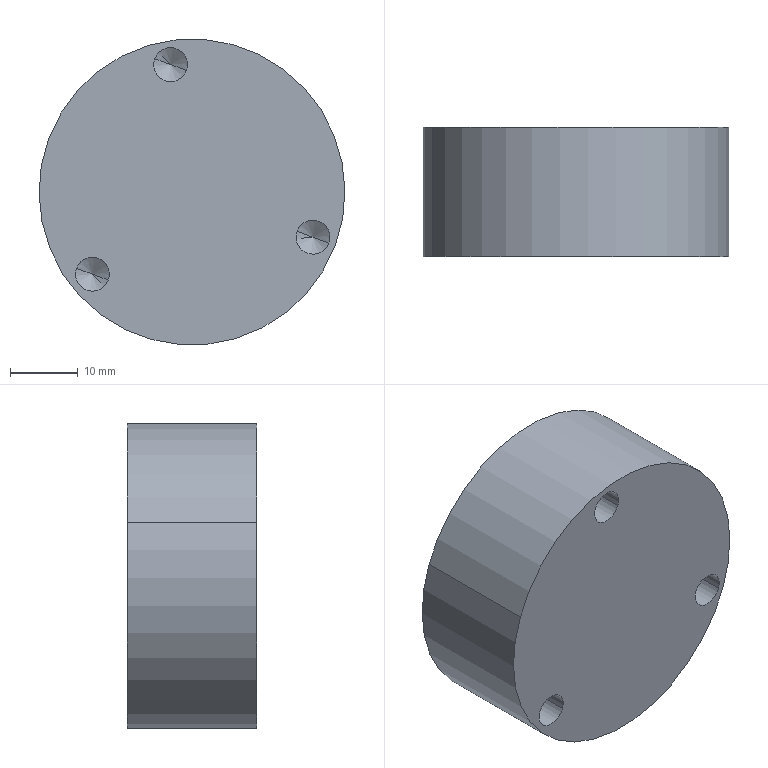Component | SolidWorks | BearingBlock-1 | 1 solid | 20 faces | box 45 x 19 x 45 mm | volume 18714 mm3 | cylinder 10 | cone 6 | spline 2 | plane 2 | commonest cylinder face diameters 5 x6 36.33 x2 45 x2
STEP:
#1=COLOUR_RGB('',0.7922,0.8196,0.9333);
#2=FILL_AREA_STYLE_COLOUR('',#1);
#3=FILL_AREA_STYLE('',(#2));
#4=SURFACE_STYLE_FILL_AREA(#3);
#5=SURFACE_SIDE_STYLE('',(#4));
#6=SURFACE_STYLE_USAGE(.BOTH.,#5);
#7=PRESENTATION_STYLE_ASSIGNMENT((#6));
#8=CARTESIAN_POINT('',(3.722,1.024,19.608));
#9=VERTEX_POINT('',#8);
#10=CARTESIAN_POINT('',(5.061,1.024,19.107));
#11=VERTEX_POINT('',#10);
#12=CARTESIAN_POINT('',(4.392,1.024,19.357));
#13=DIRECTION('',(-0.,1.,0.));
#14=DIRECTION('',(-0.9367,-0.,0.3501));
#15=AXIS2_PLACEMENT_3D('',#12,#13,#14);
#16=CIRCLE('',#15,0.7152);
#17=EDGE_CURVE('',#9,#11,#16,.T.);
#18=ORIENTED_EDGE('',*,*,#17,.T.);
#19=CARTESIAN_POINT('',(4.392,0.5906,19.357));
#20=VERTEX_POINT('',#19);
#21=CARTESIAN_POINT('',(5.061,1.024,19.107));
#22=CARTESIAN_POINT('',(4.727,0.5905,19.232));
#23=CARTESIAN_POINT('',(4.392,0.5906,19.357));
#24=B_SPLINE_CURVE_WITH_KNOTS('',2,(#21,#22,#23),.UNSPECIFIED.,.F.,.F.,(3,3),(0.06428,0.5001),.UNSPECIFIED.);
#25=EDGE_CURVE('',#11,#20,#24,.T.);
#26=ORIENTED_EDGE('',*,*,#25,.T.);
#27=CARTESIAN_POINT('',(3.722,1.024,19.608));
#28=CARTESIAN_POINT('',(4.057,0.5905,19.482));
#29=CARTESIAN_POINT('',(4.392,0.5906,19.357));
#30=B_SPLINE_CURVE_WITH_KNOTS('',2,(#27,#28,#29),.UNSPECIFIED.,.F.,.F.,(3,3),(0.06428,0.5001),.UNSPECIFIED.);
#31=EDGE_CURVE('',#9,#20,#30,.T.);
#32=ORIENTED_EDGE('',*,*,#31,.F.);
#33=EDGE_LOOP('',(#18,#26,#32));
#34=FACE_OUTER_BOUND('',#33,.T.);
#35=CARTESIAN_POINT('',(3.722,1.024,19.608));
#36=CARTESIAN_POINT('',(4.222,1.024,20.947));
#37=CARTESIAN_POINT('',(5.562,1.024,20.447));
#38=CARTESIAN_POINT('',(5.061,1.024,19.107));
#39=CARTESIAN_POINT('',(4.057,0.5905,19.482));
#40=CARTESIAN_POINT('',(4.307,0.5905,20.152));
#41=CARTESIAN_POINT('',(4.977,0.5905,19.902));
#42=CARTESIAN_POINT('',(4.727,0.5905,19.232));
#43=CARTESIAN_POINT('',(4.392,0.5906,19.357));
#44=CARTESIAN_POINT('',(4.392,0.5906,19.357));
#45=CARTESIAN_POINT('',(4.392,0.5906,19.357));
#46=CARTESIAN_POINT('',(4.392,0.5906,19.357));
#47=(BOUNDED_SURFACE()B_SPLINE_SURFACE(2,3,((#35,#36,#37,#38),(#39,#40,#41,#42),(#43,#44,#45,#46)),.UNSPECIFIED.,.F.,.F.,.F.)B_SPLINE_SURFACE_WITH_KNOTS((3,3),(4,4),(0.06428,0.5001),(0.,1.),.UNSPECIFIED.)GEOMETRIC_REPRESENTATION_ITEM()RATIONAL_B_SPLINE_SURFACE(((1.,0.3333,0.3333,1.),(1.,0.3333,0.3333,1.),(1.,0.3333,0.3333,1.)))REPRESENTATION_ITEM('')SURFACE());
#48=ADVANCED_FACE('',(#34),#47,.F.);
#49=CARTESIAN_POINT('',(4.176,0.8661,20.129));
#50=VERTEX_POINT('',#49);
#51=CARTESIAN_POINT('',(4.36,0.8661,20.06));
#52=VERTEX_POINT('',#51);
#53=CARTESIAN_POINT('',(4.268,0.8661,20.095));
#54=DIRECTION('',(0.,-1.,-0.));
#55=DIRECTION('',(0.9367,0.,-0.3501));
#56=AXIS2_PLACEMENT_3D('',#53,#54,#55);
#57=CIRCLE('',#56,0.09843);
#58=EDGE_CURVE('',#50,#52,#57,.T.);
#59=ORIENTED_EDGE('',*,*,#58,.F.);
#60=CARTESIAN_POINT('',(4.176,0.4724,20.129));
#61=VERTEX_POINT('',#60);
#62=CARTESIAN_POINT('',(4.176,0.4724,20.129));
#63=DIRECTION('',(0.,-1.,-0.));
#64=VECTOR('',#63,39.37);
#65=LINE('',#62,#64);
#66=EDGE_CURVE('',#50,#61,#65,.T.);
#67=ORIENTED_EDGE('',*,*,#66,.T.);
#68=CARTESIAN_POINT('',(4.36,0.4724,20.06));
#69=VERTEX_POINT('',#68);
#70=CARTESIAN_POINT('',(4.268,0.4724,20.095));
#71=DIRECTION('',(0.,-1.,-0.));
#72=DIRECTION('',(0.9367,0.,-0.3501));
#73=AXIS2_PLACEMENT_3D('',#70,#71,#72);
#74=CIRCLE('',#73,0.09843);
#75=EDGE_CURVE('',#61,#69,#74,.T.);
#76=ORIENTED_EDGE('',*,*,#75,.T.);
#77=CARTESIAN_POINT('',(4.36,0.4724,20.06));
#78=DIRECTION('',(0.,-1.,-0.));
#79=VECTOR('',#78,39.37);
#80=LINE('',#77,#79);
#81=EDGE_CURVE('',#52,#69,#80,.T.);
#82=ORIENTED_EDGE('',*,*,#81,.F.);
#83=EDGE_LOOP('',(#59,#67,#76,#82));
#84=FACE_OUTER_BOUND('',#83,.T.);
#85=CARTESIAN_POINT('',(4.268,0.4724,20.095));
#86=DIRECTION('',(0.,-1.,-0.));
#87=DIRECTION('',(0.9367,0.,-0.3501));
#88=AXIS2_PLACEMENT_3D('',#85,#86,#87);
#89=CYLINDRICAL_SURFACE('',#88,0.09843);
#90=ADVANCED_FACE('',(#84),#89,.F.);
#91=CARTESIAN_POINT('',(4.268,0.9253,20.095));
#92=VERTEX_POINT('',#91);
#93=CARTESIAN_POINT('',(4.36,0.8661,20.06));
#94=DIRECTION('',(0.8029,-0.515,-0.3001));
#95=VECTOR('',#94,39.37);
#96=LINE('',#93,#95);
#97=EDGE_CURVE('',#92,#52,#96,.T.);
#98=ORIENTED_EDGE('',*,*,#97,.F.);
#99=CARTESIAN_POINT('',(4.176,0.8661,20.129));
#100=DIRECTION('',(-0.8029,-0.515,0.3001));
#101=VECTOR('',#100,39.37);
#102=LINE('',#99,#101);
#103=EDGE_CURVE('',#92,#50,#102,.T.);
#104=ORIENTED_EDGE('',*,*,#103,.T.);
#105=ORIENTED_EDGE('',*,*,#58,.T.);
#106=EDGE_LOOP('',(#98,#104,#105));
#107=FACE_OUTER_BOUND('',#106,.T.);
#108=CARTESIAN_POINT('',(4.268,0.8661,20.095));
#109=DIRECTION('',(0.,-1.,-0.));
#110=DIRECTION('',(0.9367,0.,-0.3501));
#111=AXIS2_PLACEMENT_3D('',#108,#109,#110);
#112=CONICAL_SURFACE('',#111,0.09843,1.03);
#113=ADVANCED_FACE('',(#107),#112,.F.);
#114=CARTESIAN_POINT('',(5.,0.8661,19.13));
#115=VERTEX_POINT('',#114);
#116=CARTESIAN_POINT('',(5.184,0.8661,19.061));
#117=VERTEX_POINT('',#116);
#118=CARTESIAN_POINT('',(5.092,0.8661,19.095));
#119=DIRECTION('',(0.,-1.,-0.));
#120=DIRECTION('',(0.9367,0.,-0.3501));
#121=AXIS2_PLACEMENT_3D('',#118,#119,#120);
#122=CIRCLE('',#121,0.09843);
#123=EDGE_CURVE('',#115,#117,#122,.T.);
#124=ORIENTED_EDGE('',*,*,#123,.F.);
#125=CARTESIAN_POINT('',(5.,0.4724,19.13));
#126=VERTEX_POINT('',#125);
#127=CARTESIAN_POINT('',(5.,0.4724,19.13));
#128=DIRECTION('',(0.,-1.,-0.));
#129=VECTOR('',#128,39.37);
#130=LINE('',#127,#129);
#131=EDGE_CURVE('',#115,#126,#130,.T.);
#132=ORIENTED_EDGE('',*,*,#131,.T.);
#133=CARTESIAN_POINT('',(5.184,0.4724,19.061));
#134=VERTEX_POINT('',#133);
#135=CARTESIAN_POINT('',(5.092,0.4724,19.095));
#136=DIRECTION('',(0.,-1.,-0.));
#137=DIRECTION('',(0.9367,0.,-0.3501));
#138=AXIS2_PLACEMENT_3D('',#135,#136,#137);
#139=CIRCLE('',#138,0.09843);
#140=EDGE_CURVE('',#126,#134,#139,.T.);
#141=ORIENTED_EDGE('',*,*,#140,.T.);
#142=CARTESIAN_POINT('',(5.184,0.4724,19.061));
#143=DIRECTION('',(0.,-1.,-0.));
#144=VECTOR('',#143,39.37);
#145=LINE('',#142,#144);
#146=EDGE_CURVE('',#117,#134,#145,.T.);
#147=ORIENTED_EDGE('',*,*,#146,.F.);
#148=EDGE_LOOP('',(#124,#132,#141,#147));
#149=FACE_OUTER_BOUND('',#148,.T.);
#150=CARTESIAN_POINT('',(5.092,0.4724,19.095));
#151=DIRECTION('',(0.,-1.,-0.));
#152=DIRECTION('',(0.9367,0.,-0.3501));
#153=AXIS2_PLACEMENT_3D('',#150,#151,#152);
#154=CYLINDRICAL_SURFACE('',#153,0.09843);
#155=ADVANCED_FACE('',(#149),#154,.F.);
#156=CARTESIAN_POINT('',(5.092,0.9253,19.095));
#157=VERTEX_POINT('',#156);
#158=CARTESIAN_POINT('',(5.184,0.8661,19.061));
#159=DIRECTION('',(0.8029,-0.515,-0.3001));
#160=VECTOR('',#159,39.37);
#161=LINE('',#158,#160);
#162=EDGE_CURVE('',#157,#117,#161,.T.);
#163=ORIENTED_EDGE('',*,*,#162,.F.);
#164=CARTESIAN_POINT('',(5.,0.8661,19.13));
#165=DIRECTION('',(-0.8029,-0.515,0.3001));
#166=VECTOR('',#165,39.37);
#167=LINE('',#164,#166);
#168=EDGE_CURVE('',#157,#115,#167,.T.);
#169=ORIENTED_EDGE('',*,*,#168,.T.);
#170=ORIENTED_EDGE('',*,*,#123,.T.);
#171=EDGE_LOOP('',(#163,#169,#170));
#172=FACE_OUTER_BOUND('',#171,.T.);
#173=CARTESIAN_POINT('',(5.092,0.8661,19.095));
#174=DIRECTION('',(0.,-1.,-0.));
#175=DIRECTION('',(0.9367,0.,-0.3501));
#176=AXIS2_PLACEMENT_3D('',#173,#174,#175);
#177=CONICAL_SURFACE('',#176,0.09843,1.03);
#178=ADVANCED_FACE('',(#172),#177,.F.);
#179=CARTESIAN_POINT('',(3.722,0.8661,18.916));
#180=VERTEX_POINT('',#179);
#181=CARTESIAN_POINT('',(3.907,0.8661,18.847));
#182=VERTEX_POINT('',#181);
#183=CARTESIAN_POINT('',(3.814,0.8661,18.881));
#184=DIRECTION('',(0.,-1.,-0.));
#185=DIRECTION('',(0.9367,0.,-0.3501));
#186=AXIS2_PLACEMENT_3D('',#183,#184,#185);
#187=CIRCLE('',#186,0.09843);
#188=EDGE_CURVE('',#180,#182,#187,.T.);
#189=ORIENTED_EDGE('',*,*,#188,.F.);
#190=CARTESIAN_POINT('',(3.722,0.4724,18.916));
#191=VERTEX_POINT('',#190);
#192=CARTESIAN_POINT('',(3.722,0.4724,18.916));
#193=DIRECTION('',(0.,-1.,-0.));
#194=VECTOR('',#193,39.37);
#195=LINE('',#192,#194);
#196=EDGE_CURVE('',#180,#191,#195,.T.);
#197=ORIENTED_EDGE('',*,*,#196,.T.);
#198=CARTESIAN_POINT('',(3.907,0.4724,18.847));
#199=VERTEX_POINT('',#198);
#200=CARTESIAN_POINT('',(3.814,0.4724,18.881));
#201=DIRECTION('',(0.,-1.,-0.));
#202=DIRECTION('',(0.9367,0.,-0.3501));
#203=AXIS2_PLACEMENT_3D('',#200,#201,#202);
#204=CIRCLE('',#203,0.09843);
#205=EDGE_CURVE('',#191,#199,#204,.T.);
#206=ORIENTED_EDGE('',*,*,#205,.T.);
#207=CARTESIAN_POINT('',(3.907,0.4724,18.847));
#208=DIRECTION('',(0.,-1.,-0.));
#209=VECTOR('',#208,39.37);
#210=LINE('',#207,#209);
#211=EDGE_CURVE('',#182,#199,#210,.T.);
#212=ORIENTED_EDGE('',*,*,#211,.F.);
#213=EDGE_LOOP('',(#189,#197,#206,#212));
#214=FACE_OUTER_BOUND('',#213,.T.);
#215=CARTESIAN_POINT('',(3.814,0.4724,18.881));
#216=DIRECTION('',(0.,-1.,-0.));
#217=DIRECTION('',(0.9367,0.,-0.3501));
#218=AXIS2_PLACEMENT_3D('',#215,#216,#217);
#219=CYLINDRICAL_SURFACE('',#218,0.09843);
#220=ADVANCED_FACE('',(#214),#219,.F.);
#221=CARTESIAN_POINT('',(3.814,0.9253,18.881));
#222=VERTEX_POINT('',#221);
#223=CARTESIAN_POINT('',(3.907,0.8661,18.847));
#224=DIRECTION('',(0.8029,-0.515,-0.3001));
#225=VECTOR('',#224,39.37);
#226=LINE('',#223,#225);
#227=EDGE_CURVE('',#222,#182,#226,.T.);
#228=ORIENTED_EDGE('',*,*,#227,.F.);
#229=CARTESIAN_POINT('',(3.722,0.8661,18.916));
#230=DIRECTION('',(-0.8029,-0.515,0.3001));
#231=VECTOR('',#230,39.37);
#232=LINE('',#229,#231);
#233=EDGE_CURVE('',#222,#180,#232,.T.);
#234=ORIENTED_EDGE('',*,*,#233,.T.);
#235=ORIENTED_EDGE('',*,*,#188,.T.);
#236=EDGE_LOOP('',(#228,#234,#235));
#237=FACE_OUTER_BOUND('',#236,.T.);
#238=CARTESIAN_POINT('',(3.814,0.8661,18.881));
#239=DIRECTION('',(0.,-1.,-0.));
#240=DIRECTION('',(0.9367,0.,-0.3501));
#241=AXIS2_PLACEMENT_3D('',#238,#239,#240);
#242=CONICAL_SURFACE('',#241,0.09843,1.03);
#243=ADVANCED_FACE('',(#237),#242,.F.);
#244=CARTESIAN_POINT('',(4.392,1.024,19.357));
#245=DIRECTION('',(-0.,1.,0.));
#246=DIRECTION('',(-0.9367,-0.,0.3501));
#247=AXIS2_PLACEMENT_3D('',#244,#245,#246);
#248=CIRCLE('',#247,0.7152);
#249=EDGE_CURVE('',#11,#9,#248,.T.);
#250=ORIENTED_EDGE('',*,*,#249,.F.);
#251=CARTESIAN_POINT('',(5.061,1.22,19.107));
#252=VERTEX_POINT('',#251);
#253=CARTESIAN_POINT('',(5.061,1.024,19.107));
#254=DIRECTION('',(-0.,1.,0.));
#255=VECTOR('',#254,39.37);
#256=LINE('',#253,#255);
#257=EDGE_CURVE('',#11,#252,#256,.T.);
#258=ORIENTED_EDGE('',*,*,#257,.T.);
#259=CARTESIAN_POINT('',(3.722,1.22,19.608));
#260=VERTEX_POINT('',#259);
#261=CARTESIAN_POINT('',(4.392,1.22,19.357));
#262=DIRECTION('',(-0.,1.,0.));
#263=DIRECTION('',(-0.9367,-0.,0.3501));
#264=AXIS2_PLACEMENT_3D('',#261,#262,#263);
#265=CIRCLE('',#264,0.7152);
#266=EDGE_CURVE('',#252,#260,#265,.T.);
#267=ORIENTED_EDGE('',*,*,#266,.T.);
#268=CARTESIAN_POINT('',(3.722,1.024,19.608));
#269=DIRECTION('',(-0.,1.,0.));
#270=VECTOR('',#269,39.37);
#271=LINE('',#268,#270);
#272=EDGE_CURVE('',#9,#260,#271,.T.);
#273=ORIENTED_EDGE('',*,*,#272,.F.);
#274=EDGE_LOOP('',(#250,#258,#267,#273));
#275=FACE_OUTER_BOUND('',#274,.T.);
#276=CARTESIAN_POINT('',(4.392,1.024,19.357));
#277=DIRECTION('',(-0.,1.,0.));
#278=DIRECTION('',(-0.9367,-0.,0.3501));
#279=AXIS2_PLACEMENT_3D('',#276,#277,#278);
#280=CYLINDRICAL_SURFACE('',#279,0.7152);
#281=ADVANCED_FACE('',(#275),#280,.F.);
#282=CARTESIAN_POINT('',(5.221,1.22,19.047));
#283=VERTEX_POINT('',#282);
#284=CARTESIAN_POINT('',(3.562,1.22,19.667));
#285=VERTEX_POINT('',#284);
#286=CARTESIAN_POINT('',(4.392,1.22,19.357));
#287=DIRECTION('',(0.,-1.,-0.));
#288=DIRECTION('',(0.9367,0.,-0.3501));
#289=AXIS2_PLACEMENT_3D('',#286,#287,#288);
#290=CIRCLE('',#289,0.8858);
#291=EDGE_CURVE('',#283,#285,#290,.T.);
#292=ORIENTED_EDGE('',*,*,#291,.T.);
#293=CARTESIAN_POINT('',(3.562,0.4724,19.667));
#294=VERTEX_POINT('',#293);
#295=CARTESIAN_POINT('',(3.562,1.22,19.667));
#296=DIRECTION('',(0.,-1.,-0.));
#297=VECTOR('',#296,39.37);
#298=LINE('',#295,#297);
#299=EDGE_CURVE('',#285,#294,#298,.T.);
#300=ORIENTED_EDGE('',*,*,#299,.T.);
#301=CARTESIAN_POINT('',(5.221,0.4724,19.047));
#302=VERTEX_POINT('',#301);
#303=CARTESIAN_POINT('',(4.392,0.4724,19.357));
#304=DIRECTION('',(0.,-1.,-0.));
#305=DIRECTION('',(0.9367,0.,-0.3501));
#306=AXIS2_PLACEMENT_3D('',#303,#304,#305);
#307=CIRCLE('',#306,0.8858);
#308=EDGE_CURVE('',#302,#294,#307,.T.);
#309=ORIENTED_EDGE('',*,*,#308,.F.);
#310=CARTESIAN_POINT('',(5.221,1.22,19.047));
#311=DIRECTION('',(0.,-1.,-0.));
#312=VECTOR('',#311,39.37);
#313=LINE('',#310,#312);
#314=EDGE_CURVE('',#283,#302,#313,.T.);
#315=ORIENTED_EDGE('',*,*,#314,.F.);
#316=EDGE_LOOP('',(#292,#300,#309,#315));
#317=FACE_OUTER_BOUND('',#316,.T.);
#318=CARTESIAN_POINT('',(4.392,1.22,19.357));
#319=DIRECTION('',(0.,-1.,-0.));
#320=DIRECTION('',(0.9367,0.,-0.3501));
#321=AXIS2_PLACEMENT_3D('',#318,#319,#320);
#322=CYLINDRICAL_SURFACE('',#321,0.8858);
#323=ADVANCED_FACE('',(#317),#322,.T.);
#324=ORIENTED_EDGE('',*,*,#299,.F.);
#325=CARTESIAN_POINT('',(4.392,1.22,19.357));
#326=DIRECTION('',(0.,-1.,-0.));
#327=DIRECTION('',(0.9367,0.,-0.3501));
#328=AXIS2_PLACEMENT_3D('',#325,#326,#327);
#329=CIRCLE('',#328,0.8858);
#330=EDGE_CURVE('',#285,#283,#329,.T.);
#331=ORIENTED_EDGE('',*,*,#330,.T.);
#332=ORIENTED_EDGE('',*,*,#314,.T.);
#333=CARTESIAN_POINT('',(4.392,0.4724,19.357));
#334=DIRECTION('',(0.,-1.,-0.));
#335=DIRECTION('',(0.9367,0.,-0.3501));
#336=AXIS2_PLACEMENT_3D('',#333,#334,#335);
#337=CIRCLE('',#336,0.8858);
#338=EDGE_CURVE('',#294,#302,#337,.T.);
#339=ORIENTED_EDGE('',*,*,#338,.F.);
#340=EDGE_LOOP('',(#324,#331,#332,#339));
#341=FACE_OUTER_BOUND('',#340,.T.);
#342=CARTESIAN_POINT('',(4.392,1.22,19.357));
#343=DIRECTION('',(0.,-1.,-0.));
#344=DIRECTION('',(0.9367,0.,-0.3501));
#345=AXIS2_PLACEMENT_3D('',#342,#343,#344);
#346=CYLINDRICAL_SURFACE('',#345,0.8858);
#347=ADVANCED_FACE('',(#341),#346,.T.);
#348=CARTESIAN_POINT('',(4.392,1.22,19.357));
#349=DIRECTION('',(-0.,1.,0.));
#350=DIRECTION('',(-0.9367,-0.,0.3501));
#351=AXIS2_PLACEMENT_3D('',#348,#349,#350);
#352=CIRCLE('',#351,0.7152);
#353=EDGE_CURVE('',#260,#252,#352,.T.);
#354=ORIENTED_EDGE('',*,*,#353,.F.);
#355=ORIENTED_EDGE('',*,*,#266,.F.);
#356=EDGE_LOOP('',(#354,#355));
#357=FACE_BOUND('',#356,.T.);
#358=ORIENTED_EDGE('',*,*,#291,.F.);
#359=ORIENTED_EDGE('',*,*,#330,.F.);
#360=EDGE_LOOP('',(#358,#359));
#361=FACE_OUTER_BOUND('',#360,.T.);
#362=CARTESIAN_POINT('',(4.392,1.22,19.357));
#363=DIRECTION('',(0.,-1.,-0.));
#364=DIRECTION('',(0.9367,0.,-0.3501));
#365=AXIS2_PLACEMENT_3D('',#362,#363,#364);
#366=PLANE('',#365);
#367=ADVANCED_FACE('',(#357,#361),#366,.F.);
#368=CARTESIAN_POINT('',(4.268,0.4724,20.095));
#369=DIRECTION('',(0.,-1.,-0.));
#370=DIRECTION('',(0.9367,0.,-0.3501));
#371=AXIS2_PLACEMENT_3D('',#368,#369,#370);
#372=CIRCLE('',#371,0.09843);
#373=EDGE_CURVE('',#69,#61,#372,.T.);
#374=ORIENTED_EDGE('',*,*,#373,.F.);
#375=ORIENTED_EDGE('',*,*,#75,.F.);
#376=EDGE_LOOP('',(#374,#375));
#377=FACE_BOUND('',#376,.T.);
#378=CARTESIAN_POINT('',(5.092,0.4724,19.095));
#379=DIRECTION('',(0.,-1.,-0.));
#380=DIRECTION('',(0.9367,0.,-0.3501));
#381=AXIS2_PLACEMENT_3D('',#378,#379,#380);
#382=CIRCLE('',#381,0.09843);
#383=EDGE_CURVE('',#134,#126,#382,.T.);
#384=ORIENTED_EDGE('',*,*,#383,.F.);
#385=ORIENTED_EDGE('',*,*,#140,.F.);
#386=EDGE_LOOP('',(#384,#385));
#387=FACE_BOUND('',#386,.T.);
#388=CARTESIAN_POINT('',(3.814,0.4724,18.881));
#389=DIRECTION('',(0.,-1.,-0.));
#390=DIRECTION('',(0.9367,0.,-0.3501));
#391=AXIS2_PLACEMENT_3D('',#388,#389,#390);
#392=CIRCLE('',#391,0.09843);
#393=EDGE_CURVE('',#199,#191,#392,.T.);
#394=ORIENTED_EDGE('',*,*,#393,.F.);
#395=ORIENTED_EDGE('',*,*,#205,.F.);
#396=EDGE_LOOP('',(#394,#395));
#397=FACE_BOUND('',#396,.T.);
#398=ORIENTED_EDGE('',*,*,#308,.T.);
#399=ORIENTED_EDGE('',*,*,#338,.T.);
#400=EDGE_LOOP('',(#398,#399));
#401=FACE_OUTER_BOUND('',#400,.T.);
#402=CARTESIAN_POINT('',(4.392,0.4724,19.357));
#403=DIRECTION('',(0.,-1.,-0.));
#404=DIRECTION('',(0.9367,0.,-0.3501));
#405=AXIS2_PLACEMENT_3D('',#402,#403,#404);
#406=PLANE('',#405);
#407=ADVANCED_FACE('',(#377,#387,#397,#401),#406,.T.);
#408=ORIENTED_EDGE('',*,*,#257,.F.);
#409=ORIENTED_EDGE('',*,*,#17,.F.);
#410=ORIENTED_EDGE('',*,*,#272,.T.);
#411=ORIENTED_EDGE('',*,*,#353,.T.);
#412=EDGE_LOOP('',(#408,#409,#410,#411));
#413=FACE_OUTER_BOUND('',#412,.T.);
#414=CARTESIAN_POINT('',(4.392,1.024,19.357));
#415=DIRECTION('',(-0.,1.,0.));
#416=DIRECTION('',(-0.9367,-0.,0.3501));
#417=AXIS2_PLACEMENT_3D('',#414,#415,#416);
#418=CYLINDRICAL_SURFACE('',#417,0.7152);
#419=ADVANCED_FACE('',(#413),#418,.F.);
#420=ORIENTED_EDGE('',*,*,#25,.F.);
#421=ORIENTED_EDGE('',*,*,#249,.T.);
#422=ORIENTED_EDGE('',*,*,#31,.T.);
#423=EDGE_LOOP('',(#420,#421,#422));
#424=FACE_OUTER_BOUND('',#423,.T.);
#425=CARTESIAN_POINT('',(5.061,1.024,19.107));
#426=CARTESIAN_POINT('',(4.561,1.024,17.767));
#427=CARTESIAN_POINT('',(3.221,1.024,18.268));
#428=CARTESIAN_POINT('',(3.722,1.024,19.608));
#429=CARTESIAN_POINT('',(4.727,0.5905,19.232));
#430=CARTESIAN_POINT('',(4.476,0.5905,18.562));
#431=CARTESIAN_POINT('',(3.806,0.5905,18.812));
#432=CARTESIAN_POINT('',(4.057,0.5905,19.482));
#433=CARTESIAN_POINT('',(4.392,0.5906,19.357));
#434=CARTESIAN_POINT('',(4.392,0.5906,19.357));
#435=CARTESIAN_POINT('',(4.392,0.5906,19.357));
#436=CARTESIAN_POINT('',(4.392,0.5906,19.357));
#437=(BOUNDED_SURFACE()B_SPLINE_SURFACE(2,3,((#425,#426,#427,#428),(#429,#430,#431,#432),(#433,#434,#435,#436)),.UNSPECIFIED.,.F.,.F.,.F.)B_SPLINE_SURFACE_WITH_KNOTS((3,3),(4,4),(0.06428,0.5001),(0.,1.),.UNSPECIFIED.)GEOMETRIC_REPRESENTATION_ITEM()RATIONAL_B_SPLINE_SURFACE(((1.,0.3333,0.3333,1.),(1.,0.3333,0.3333,1.),(1.,0.3333,0.3333,1.)))REPRESENTATION_ITEM('')SURFACE());
#438=ADVANCED_FACE('',(#424),#437,.F.);
#439=ORIENTED_EDGE('',*,*,#233,.F.);
#440=ORIENTED_EDGE('',*,*,#227,.T.);
#441=CARTESIAN_POINT('',(3.814,0.8661,18.881));
#442=DIRECTION('',(0.,-1.,-0.));
#443=DIRECTION('',(0.9367,0.,-0.3501));
#444=AXIS2_PLACEMENT_3D('',#441,#442,#443);
#445=CIRCLE('',#444,0.09843);
#446=EDGE_CURVE('',#182,#180,#445,.T.);
#447=ORIENTED_EDGE('',*,*,#446,.T.);
#448=EDGE_LOOP('',(#439,#440,#447));
#449=FACE_OUTER_BOUND('',#448,.T.);
#450=CARTESIAN_POINT('',(3.814,0.8661,18.881));
#451=DIRECTION('',(0.,-1.,-0.));
#452=DIRECTION('',(0.9367,0.,-0.3501));
#453=AXIS2_PLACEMENT_3D('',#450,#451,#452);
#454=CONICAL_SURFACE('',#453,0.09843,1.03);
#455=ADVANCED_FACE('',(#449),#454,.F.);
#456=ORIENTED_EDGE('',*,*,#196,.F.);
#457=ORIENTED_EDGE('',*,*,#446,.F.);
#458=ORIENTED_EDGE('',*,*,#211,.T.);
#459=ORIENTED_EDGE('',*,*,#393,.T.);
#460=EDGE_LOOP('',(#456,#457,#458,#459));
#461=FACE_OUTER_BOUND('',#460,.T.);
#462=CARTESIAN_POINT('',(3.814,0.4724,18.881));
#463=DIRECTION('',(0.,-1.,-0.));
#464=DIRECTION('',(0.9367,0.,-0.3501));
#465=AXIS2_PLACEMENT_3D('',#462,#463,#464);
#466=CYLINDRICAL_SURFACE('',#465,0.09843);
#467=ADVANCED_FACE('',(#461),#466,.F.);
#468=ORIENTED_EDGE('',*,*,#168,.F.);
#469=ORIENTED_EDGE('',*,*,#162,.T.);
#470=CARTESIAN_POINT('',(5.092,0.8661,19.095));
#471=DIRECTION('',(0.,-1.,-0.));
#472=DIRECTION('',(0.9367,0.,-0.3501));
#473=AXIS2_PLACEMENT_3D('',#470,#471,#472);
#474=CIRCLE('',#473,0.09843);
#475=EDGE_CURVE('',#117,#115,#474,.T.);
#476=ORIENTED_EDGE('',*,*,#475,.T.);
#477=EDGE_LOOP('',(#468,#469,#476));
#478=FACE_OUTER_BOUND('',#477,.T.);
#479=CARTESIAN_POINT('',(5.092,0.8661,19.095));
#480=DIRECTION('',(0.,-1.,-0.));
#481=DIRECTION('',(0.9367,0.,-0.3501));
#482=AXIS2_PLACEMENT_3D('',#479,#480,#481);
#483=CONICAL_SURFACE('',#482,0.09843,1.03);
#484=ADVANCED_FACE('',(#478),#483,.F.);
#485=ORIENTED_EDGE('',*,*,#131,.F.);
#486=ORIENTED_EDGE('',*,*,#475,.F.);
#487=ORIENTED_EDGE('',*,*,#146,.T.);
#488=ORIENTED_EDGE('',*,*,#383,.T.);
#489=EDGE_LOOP('',(#485,#486,#487,#488));
#490=FACE_OUTER_BOUND('',#489,.T.);
#491=CARTESIAN_POINT('',(5.092,0.4724,19.095));
#492=DIRECTION('',(0.,-1.,-0.));
#493=DIRECTION('',(0.9367,0.,-0.3501));
#494=AXIS2_PLACEMENT_3D('',#491,#492,#493);
#495=CYLINDRICAL_SURFACE('',#494,0.09843);
#496=ADVANCED_FACE('',(#490),#495,.F.);
#497=ORIENTED_EDGE('',*,*,#103,.F.);
#498=ORIENTED_EDGE('',*,*,#97,.T.);
#499=CARTESIAN_POINT('',(4.268,0.8661,20.095));
#500=DIRECTION('',(0.,-1.,-0.));
#501=DIRECTION('',(0.9367,0.,-0.3501));
#502=AXIS2_PLACEMENT_3D('',#499,#500,#501);
#503=CIRCLE('',#502,0.09843);
#504=EDGE_CURVE('',#52,#50,#503,.T.);
#505=ORIENTED_EDGE('',*,*,#504,.T.);
#506=EDGE_LOOP('',(#497,#498,#505));
#507=FACE_OUTER_BOUND('',#506,.T.);
#508=CARTESIAN_POINT('',(4.268,0.8661,20.095));
#509=DIRECTION('',(0.,-1.,-0.));
#510=DIRECTION('',(0.9367,0.,-0.3501));
#511=AXIS2_PLACEMENT_3D('',#508,#509,#510);
#512=CONICAL_SURFACE('',#511,0.09843,1.03);
#513=ADVANCED_FACE('',(#507),#512,.F.);
#514=ORIENTED_EDGE('',*,*,#66,.F.);
#515=ORIENTED_EDGE('',*,*,#504,.F.);
#516=ORIENTED_EDGE('',*,*,#81,.T.);
#517=ORIENTED_EDGE('',*,*,#373,.T.);
#518=EDGE_LOOP('',(#514,#515,#516,#517));
#519=FACE_OUTER_BOUND('',#518,.T.);
#520=CARTESIAN_POINT('',(4.268,0.4724,20.095));
#521=DIRECTION('',(0.,-1.,-0.));
#522=DIRECTION('',(0.9367,0.,-0.3501));
#523=AXIS2_PLACEMENT_3D('',#520,#521,#522);
#524=CYLINDRICAL_SURFACE('',#523,0.09843);
#525=ADVANCED_FACE('',(#519),#524,.F.);
#526=CLOSED_SHELL('',(#48,#90,#113,#155,#178,#220,#243,#281,#323,#347,#367,#407,#419,#438,#455,#467,#484,#496,#513,#525));
#527=MANIFOLD_SOLID_BREP('',#526);
#528=STYLED_ITEM('',(#7),#527);
#529=PRESENTATION_LAYER_ASSIGNMENT('','',(#528));
#530=(LENGTH_UNIT()NAMED_UNIT(*)SI_UNIT($,.METRE.));
#531=LENGTH_MEASURE_WITH_UNIT(LENGTH_MEASURE(0.0254),#530);
#532=DIMENSIONAL_EXPONENTS(1.,0.,0.,0.,0.,0.,0.);
#533=(CONVERSION_BASED_UNIT('',#531)LENGTH_UNIT()NAMED_UNIT(#532));
#534=UNCERTAINTY_MEASURE_WITH_UNIT(LENGTH_MEASURE(0.00001),#533,'','');
#535=(NAMED_UNIT(*)PLANE_ANGLE_UNIT()SI_UNIT($,.RADIAN.));
#536=(NAMED_UNIT(*)SI_UNIT($,.STERADIAN.)SOLID_ANGLE_UNIT());
#537=(GEOMETRIC_REPRESENTATION_CONTEXT(3)GLOBAL_UNCERTAINTY_ASSIGNED_CONTEXT((#534))GLOBAL_UNIT_ASSIGNED_CONTEXT((#533,#535,#536))REPRESENTATION_CONTEXT('',''));
#538=MECHANICAL_DESIGN_GEOMETRIC_PRESENTATION_REPRESENTATION('',(#528),#537);
#539=CARTESIAN_POINT('',(0.,0.,0.));
#540=DIRECTION('',(0.,0.,1.));
#541=DIRECTION('',(1.,0.,0.));
#542=AXIS2_PLACEMENT_3D('',#539,#540,#541);
#543=(LENGTH_UNIT()NAMED_UNIT(*)SI_UNIT($,.METRE.));
#544=LENGTH_MEASURE_WITH_UNIT(LENGTH_MEASURE(0.0254),#543);
#545=DIMENSIONAL_EXPONENTS(1.,0.,0.,0.,0.,0.,0.);
#546=(CONVERSION_BASED_UNIT('',#544)LENGTH_UNIT()NAMED_UNIT(#545));
#547=UNCERTAINTY_MEASURE_WITH_UNIT(LENGTH_MEASURE(0.00001),#546,'','');
#548=(NAMED_UNIT(*)PLANE_ANGLE_UNIT()SI_UNIT($,.RADIAN.));
#549=(NAMED_UNIT(*)SI_UNIT($,.STERADIAN.)SOLID_ANGLE_UNIT());
#550=(GEOMETRIC_REPRESENTATION_CONTEXT(3)GLOBAL_UNCERTAINTY_ASSIGNED_CONTEXT((#547))GLOBAL_UNIT_ASSIGNED_CONTEXT((#546,#548,#549))REPRESENTATION_CONTEXT('',''));
#551=ADVANCED_BREP_SHAPE_REPRESENTATION('',(#527,#542),#550);